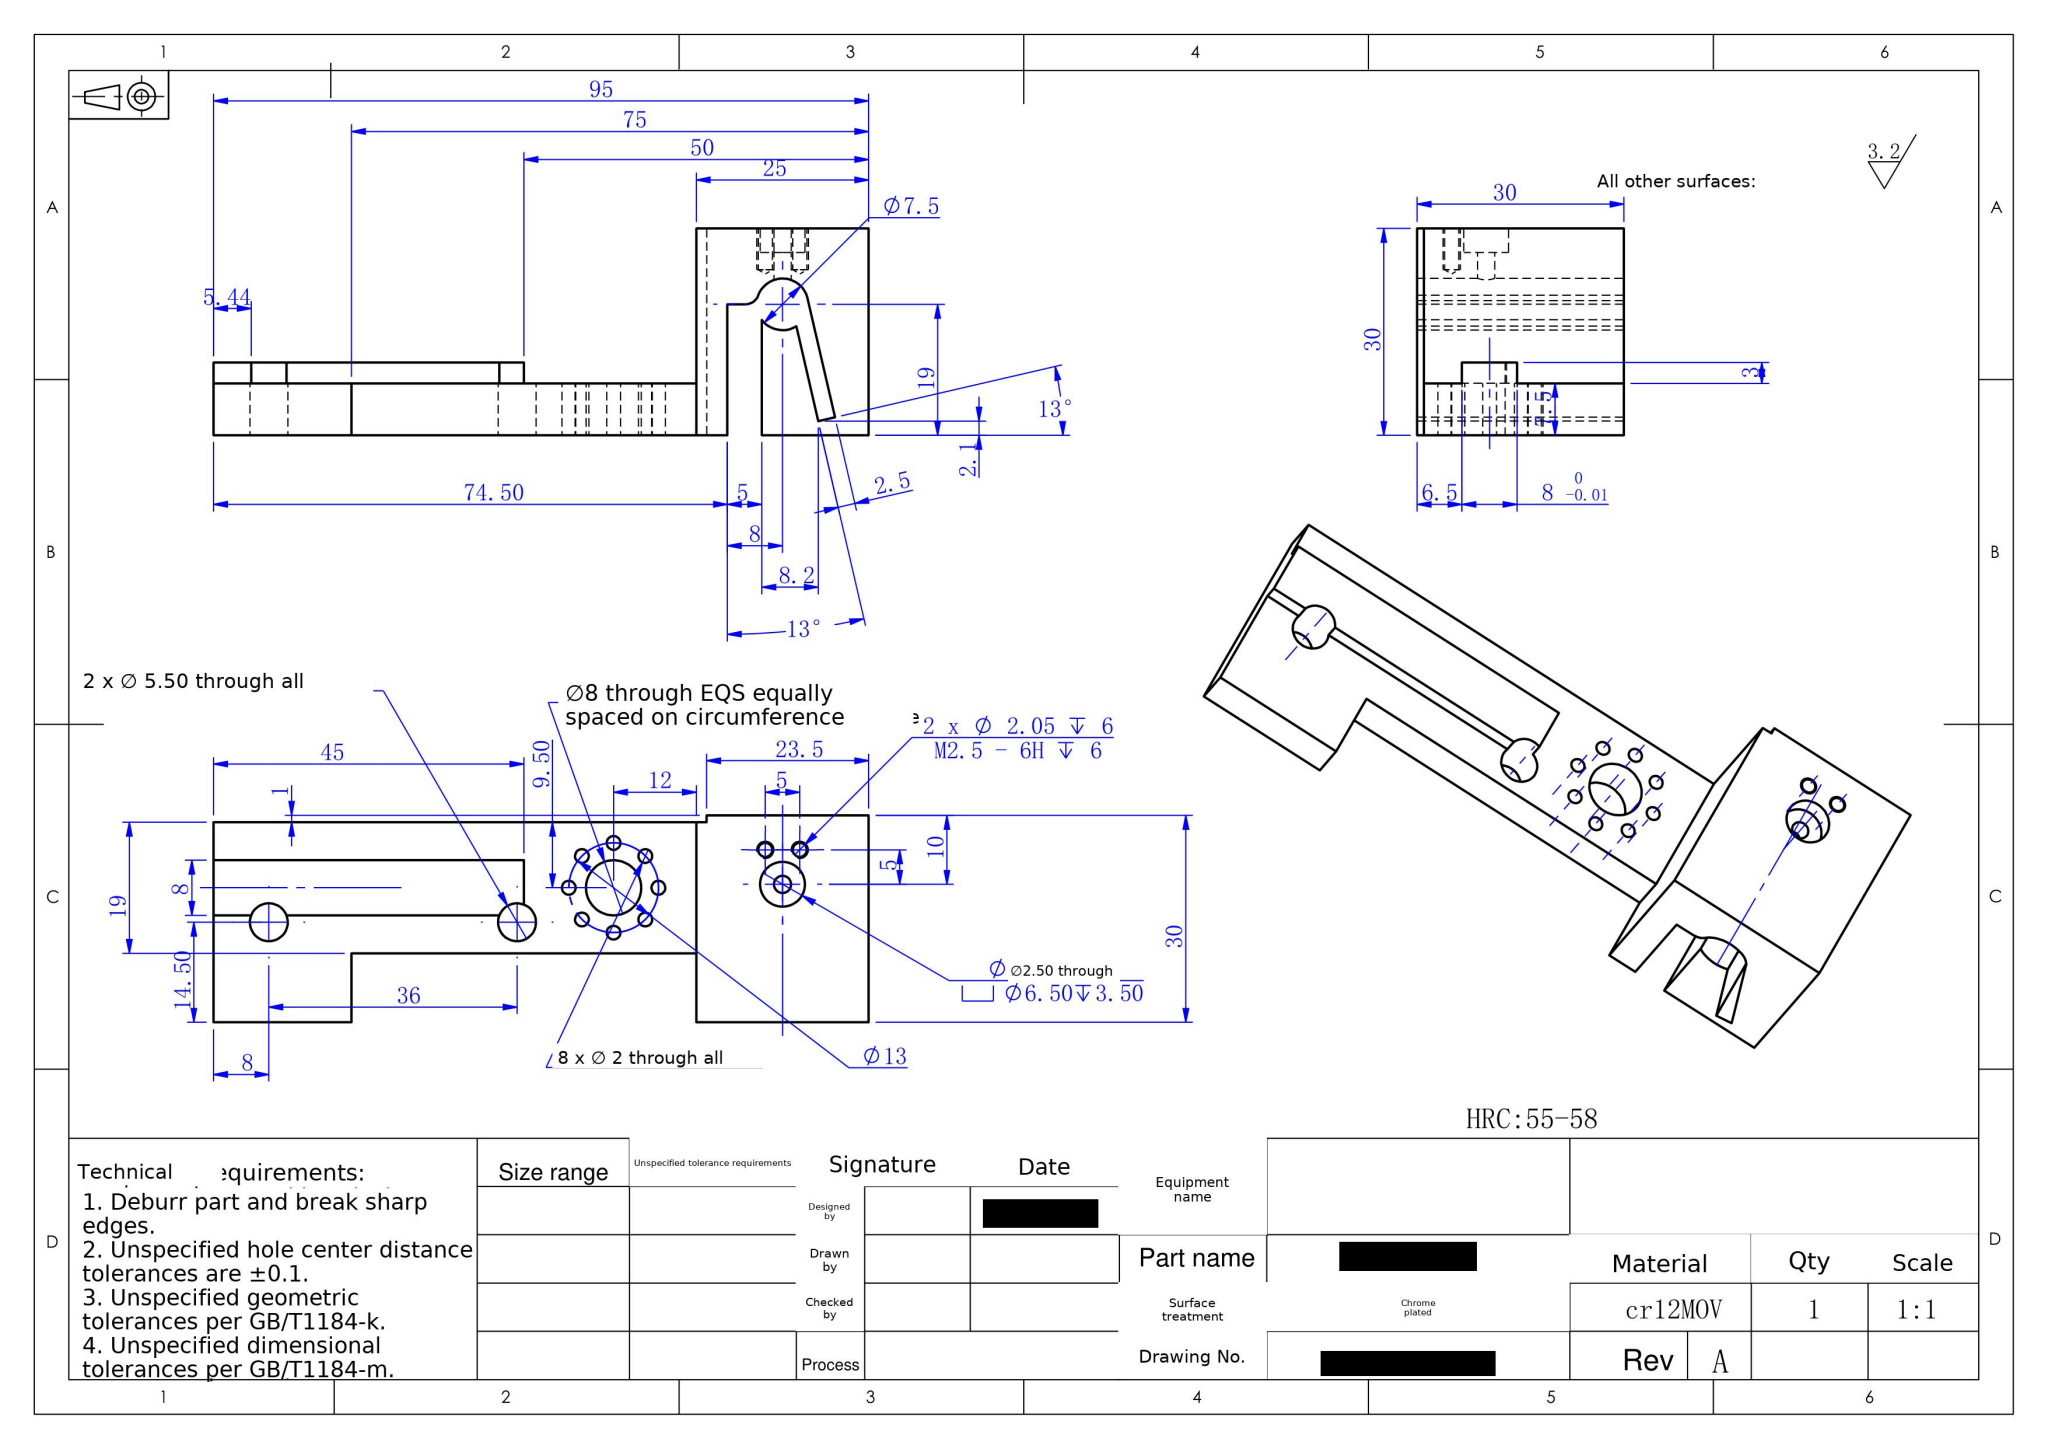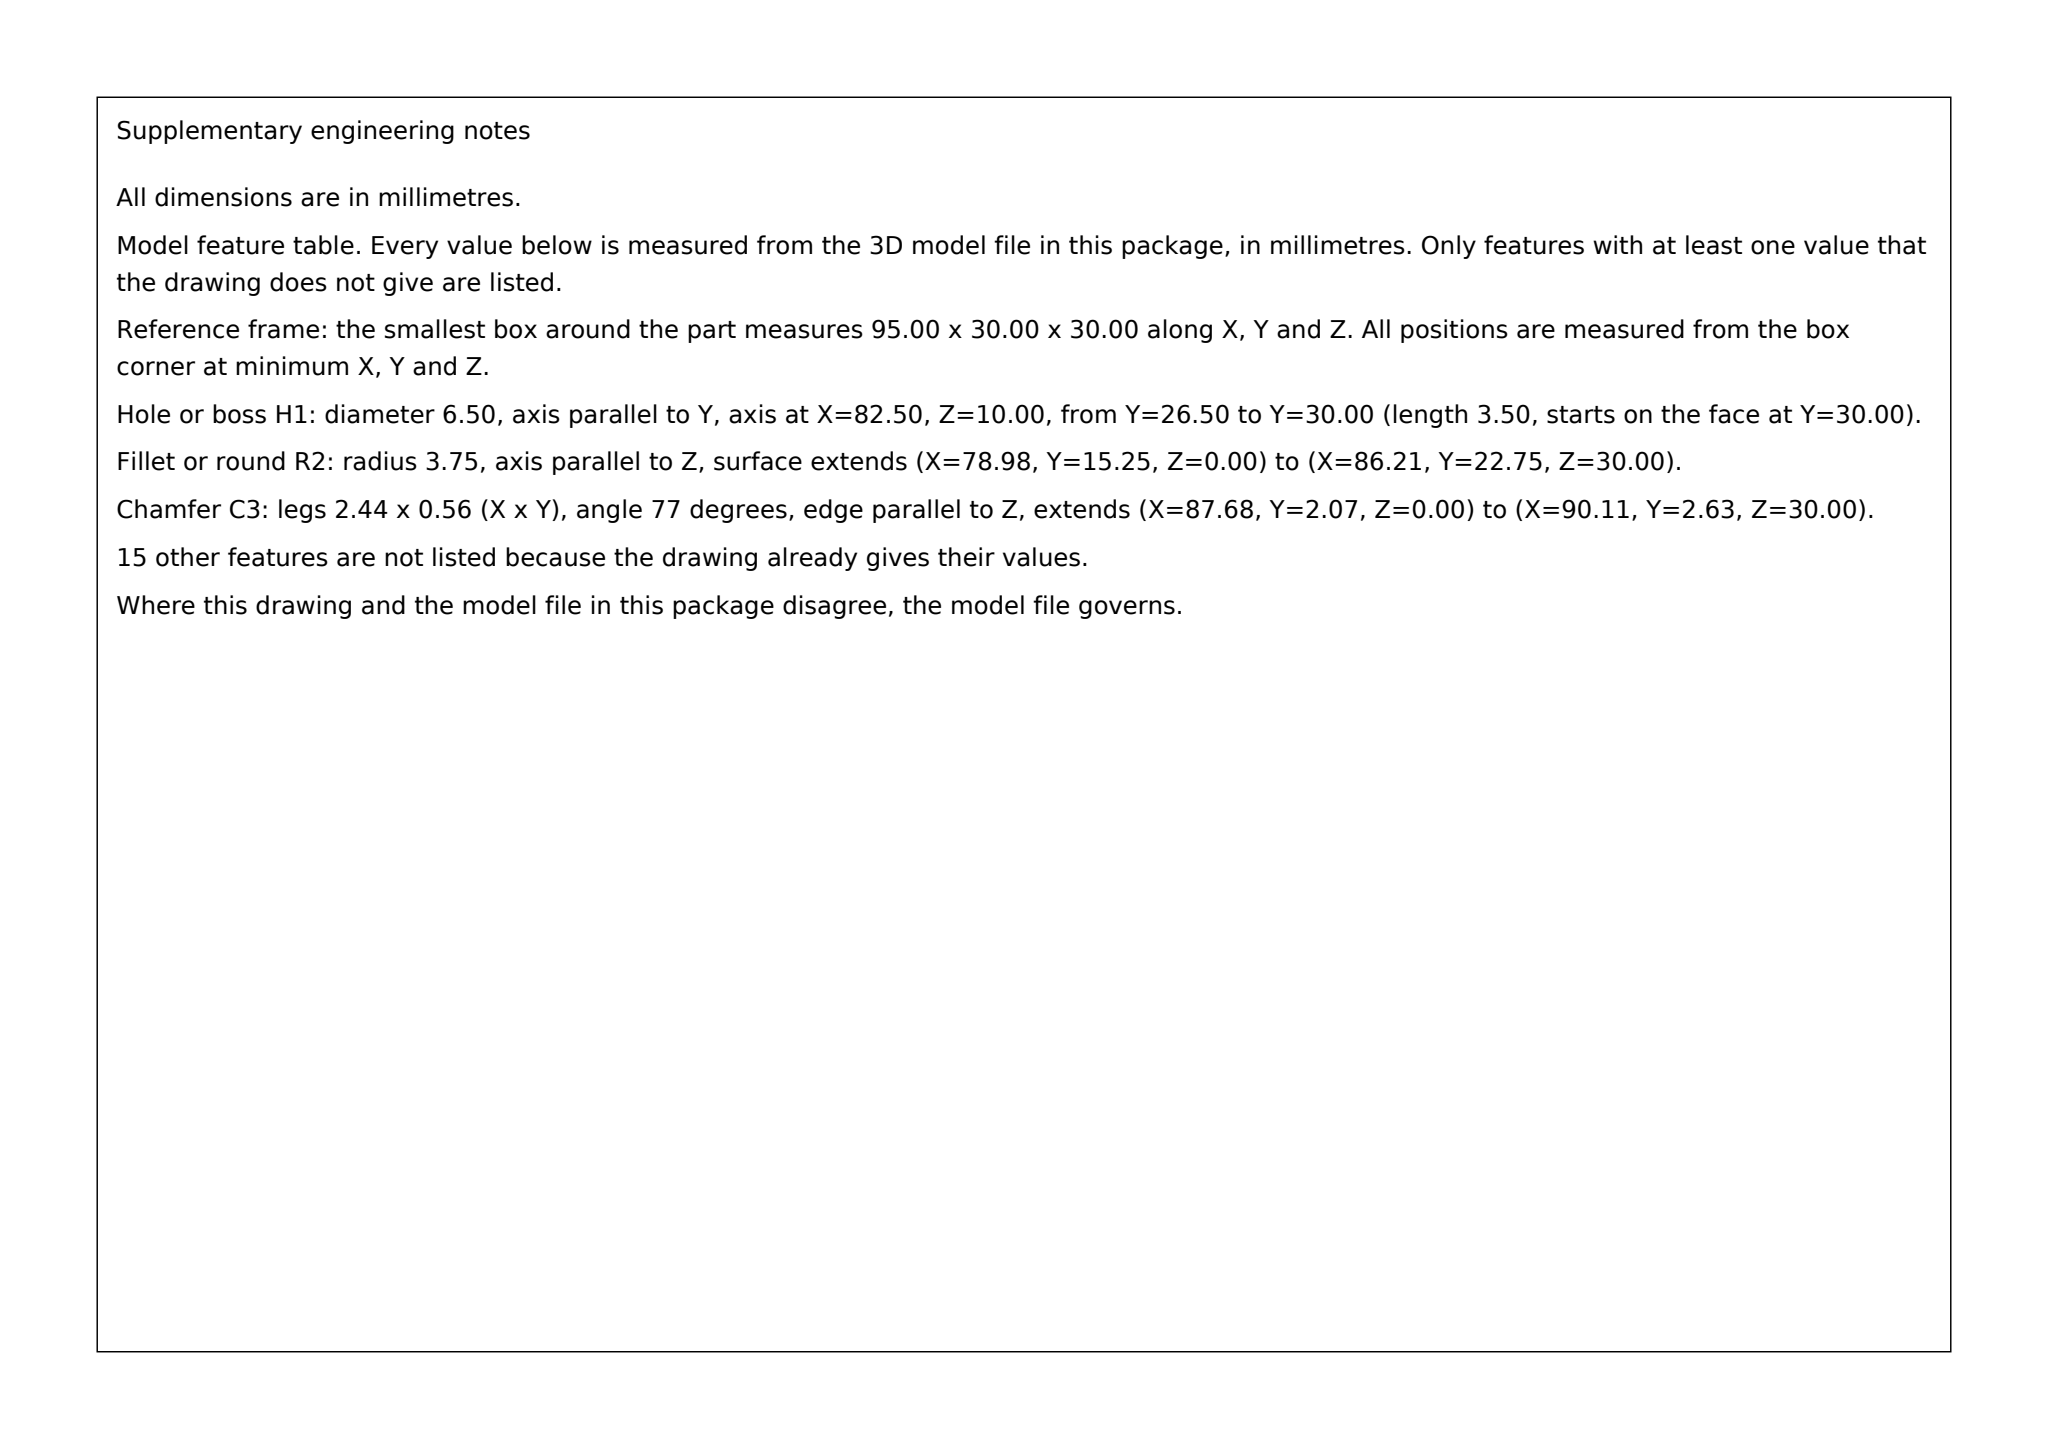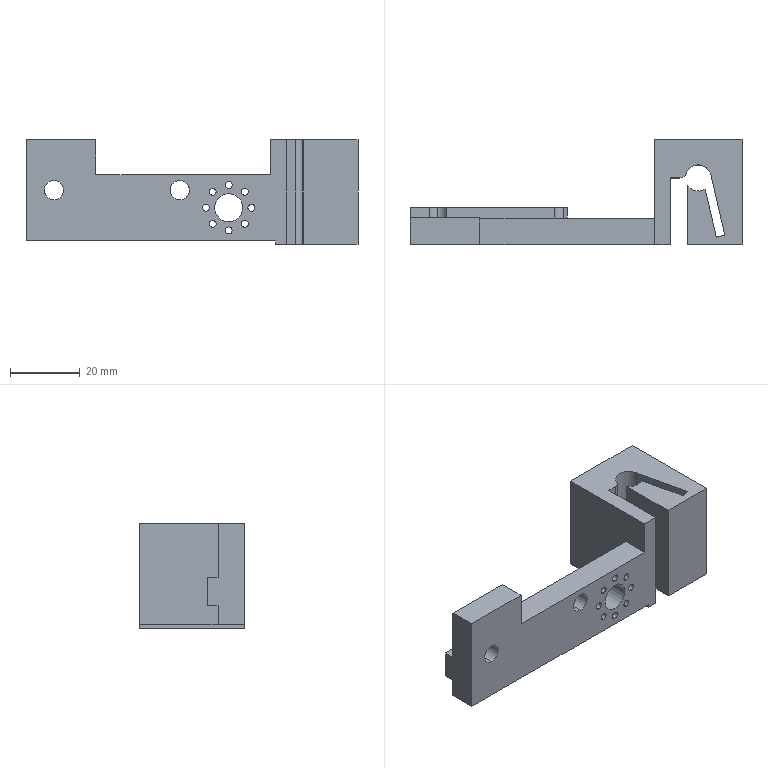Part | SolidWorks | mm | material cr12MoV | 1 solid | 63 faces | box 95 x 30 x 30 mm | volume 28662 mm3 | cylinder 33 | plane 26 | cone 4 | commonest cylinder face diameters 2 x16 2.05 x4 5.5 x4 8 x2 6.5 x2 2.5 x2 7.5 x2 4 x1